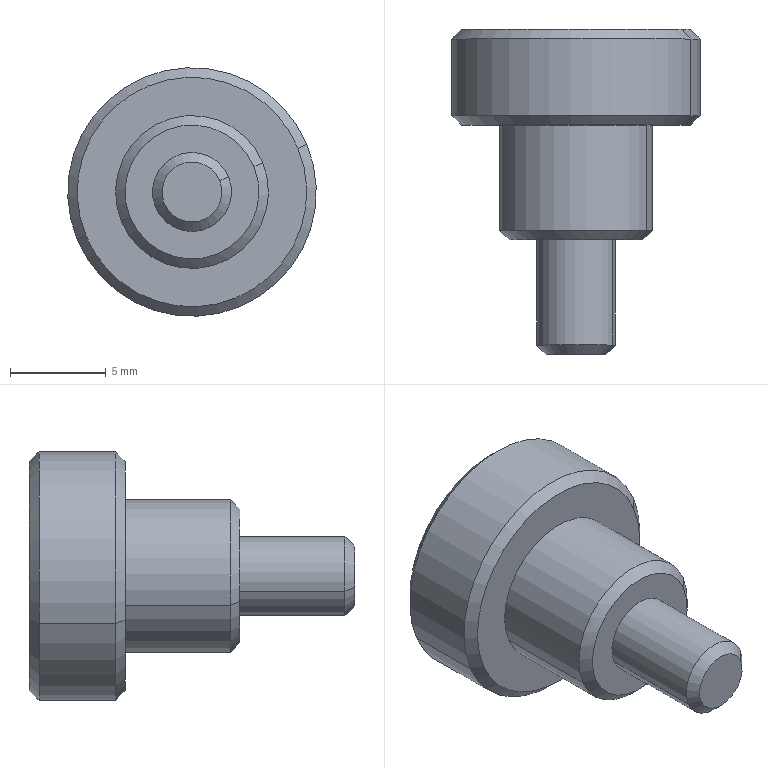Component | SolidWorks | BearingLiftingModule-1_CylinderLiftingModule-1_CHEN123-AA-26-1 | 1 solid | 18 faces | box 13 x 17 x 13 mm | volume 1031 mm3 | cone 8 | cylinder 6 | plane 4 | commonest cylinder face diameters 4.134 x2 8 x2 13 x2
build123d program:
from build123d import *

# Parameters (mm, degrees)
SKETCH1_R           = 6.5
BOSS_EXTRUDE1_DEPTH = 5
SKETCH2_R           = 4
BOSS_EXTRUDE2_DEPTH = 6
SKETCH3_R           = 2.067
BOSS_EXTRUDE3_DEPTH = 6
CHAMFER1_SIZE       = 0.5


with BuildPart() as part:
    # Sketch1 → Boss-Extrude1 (new body)
    with BuildSketch(Plane.XY):
        Circle(SKETCH1_R)
    extrude(amount=BOSS_EXTRUDE1_DEPTH)

    # Sketch2 → Boss-Extrude2 (add)
    with BuildSketch(Plane.XY.offset(5)):
        Circle(SKETCH2_R)
    extrude(amount=BOSS_EXTRUDE2_DEPTH)

    # Sketch3 → Boss-Extrude3 (add)
    with BuildSketch(Plane.XY.offset(11)):
        Circle(SKETCH3_R)
    extrude(amount=BOSS_EXTRUDE3_DEPTH)

    # Chamfer1
    chamfer1_edges = [part.edges().sort_by_distance(p)[0] for p in [
        (-2.067, 0, 17),
        (-6.5, 0, 0),
        (-6.5, 0, 5),
        (-4, 0, 11),
    ]]
    chamfer(chamfer1_edges, length=CHAMFER1_SIZE)


solid = part.part

# Placed as in the assembly
solid = solid.moved(Location((69.999, -35.699, 30), (90, 0, 0)))
STEP:
#1=COLOUR_RGB('',0.7922,0.8196,0.9333);
#2=FILL_AREA_STYLE_COLOUR('',#1);
#3=FILL_AREA_STYLE('',(#2));
#4=SURFACE_STYLE_FILL_AREA(#3);
#5=SURFACE_SIDE_STYLE('',(#4));
#6=SURFACE_STYLE_USAGE(.BOTH.,#5);
#7=PRESENTATION_STYLE_ASSIGNMENT((#6));
#8=CARTESIAN_POINT('',(2.538,-1.405,1.091));
#9=VERTEX_POINT('',#8);
#10=CARTESIAN_POINT('',(2.974,-1.405,1.271));
#11=VERTEX_POINT('',#10);
#12=CARTESIAN_POINT('',(2.756,-1.405,1.181));
#13=DIRECTION('',(-0.,1.,-0.));
#14=DIRECTION('',(0.9242,0.,0.3818));
#15=AXIS2_PLACEMENT_3D('',#12,#13,#14);
#16=CIRCLE('',#15,0.2362);
#17=EDGE_CURVE('',#9,#11,#16,.T.);
#18=ORIENTED_EDGE('',*,*,#17,.F.);
#19=CARTESIAN_POINT('',(2.519,-1.425,1.083));
#20=VERTEX_POINT('',#19);
#21=CARTESIAN_POINT('',(2.519,-1.425,1.083));
#22=DIRECTION('',(-0.6535,-0.7071,-0.27));
#23=VECTOR('',#22,39.37);
#24=LINE('',#21,#23);
#25=EDGE_CURVE('',#9,#20,#24,.T.);
#26=ORIENTED_EDGE('',*,*,#25,.T.);
#27=CARTESIAN_POINT('',(2.992,-1.425,1.279));
#28=VERTEX_POINT('',#27);
#29=CARTESIAN_POINT('',(2.756,-1.425,1.181));
#30=DIRECTION('',(0.,-1.,0.));
#31=DIRECTION('',(0.9242,0.,0.3818));
#32=AXIS2_PLACEMENT_3D('',#29,#30,#31);
#33=CIRCLE('',#32,0.2559);
#34=EDGE_CURVE('',#28,#20,#33,.T.);
#35=ORIENTED_EDGE('',*,*,#34,.F.);
#36=CARTESIAN_POINT('',(2.992,-1.425,1.279));
#37=DIRECTION('',(0.6535,-0.7071,0.27));
#38=VECTOR('',#37,39.37);
#39=LINE('',#36,#38);
#40=EDGE_CURVE('',#11,#28,#39,.T.);
#41=ORIENTED_EDGE('',*,*,#40,.F.);
#42=EDGE_LOOP('',(#18,#26,#35,#41));
#43=FACE_OUTER_BOUND('',#42,.T.);
#44=CARTESIAN_POINT('',(2.756,-1.425,1.181));
#45=DIRECTION('',(0.,-1.,0.));
#46=DIRECTION('',(0.9242,0.,0.3818));
#47=AXIS2_PLACEMENT_3D('',#44,#45,#46);
#48=CONICAL_SURFACE('',#47,0.2559,0.7854);
#49=ADVANCED_FACE('',(#43),#48,.T.);
#50=CARTESIAN_POINT('',(2.813,-2.075,1.205));
#51=VERTEX_POINT('',#50);
#52=CARTESIAN_POINT('',(2.699,-2.075,1.158));
#53=VERTEX_POINT('',#52);
#54=CARTESIAN_POINT('',(2.756,-2.075,1.181));
#55=DIRECTION('',(0.,-1.,0.));
#56=DIRECTION('',(0.9242,0.,0.3818));
#57=AXIS2_PLACEMENT_3D('',#54,#55,#56);
#58=CIRCLE('',#57,0.06169);
#59=EDGE_CURVE('',#51,#53,#58,.T.);
#60=ORIENTED_EDGE('',*,*,#59,.F.);
#61=CARTESIAN_POINT('',(2.831,-2.055,1.212));
#62=VERTEX_POINT('',#61);
#63=CARTESIAN_POINT('',(2.813,-2.075,1.205));
#64=DIRECTION('',(0.6535,0.7071,0.27));
#65=VECTOR('',#64,39.37);
#66=LINE('',#63,#65);
#67=EDGE_CURVE('',#51,#62,#66,.T.);
#68=ORIENTED_EDGE('',*,*,#67,.T.);
#69=CARTESIAN_POINT('',(2.681,-2.055,1.15));
#70=VERTEX_POINT('',#69);
#71=CARTESIAN_POINT('',(2.756,-2.055,1.181));
#72=DIRECTION('',(-0.,1.,-0.));
#73=DIRECTION('',(0.9242,0.,0.3818));
#74=AXIS2_PLACEMENT_3D('',#71,#72,#73);
#75=CIRCLE('',#74,0.08138);
#76=EDGE_CURVE('',#70,#62,#75,.T.);
#77=ORIENTED_EDGE('',*,*,#76,.F.);
#78=CARTESIAN_POINT('',(2.699,-2.075,1.158));
#79=DIRECTION('',(-0.6535,0.7071,-0.27));
#80=VECTOR('',#79,39.37);
#81=LINE('',#78,#80);
#82=EDGE_CURVE('',#53,#70,#81,.T.);
#83=ORIENTED_EDGE('',*,*,#82,.F.);
#84=EDGE_LOOP('',(#60,#68,#77,#83));
#85=FACE_OUTER_BOUND('',#84,.T.);
#86=CARTESIAN_POINT('',(2.756,-2.075,1.181));
#87=DIRECTION('',(-0.,1.,-0.));
#88=DIRECTION('',(-0.9242,0.,-0.3818));
#89=AXIS2_PLACEMENT_3D('',#86,#87,#88);
#90=CONICAL_SURFACE('',#89,0.06169,0.7854);
#91=ADVANCED_FACE('',(#85),#90,.T.);
#92=CARTESIAN_POINT('',(2.883,-1.839,1.234));
#93=VERTEX_POINT('',#92);
#94=CARTESIAN_POINT('',(2.629,-1.839,1.128));
#95=VERTEX_POINT('',#94);
#96=CARTESIAN_POINT('',(2.756,-1.839,1.181));
#97=DIRECTION('',(0.,-1.,0.));
#98=DIRECTION('',(0.9242,0.,0.3818));
#99=AXIS2_PLACEMENT_3D('',#96,#97,#98);
#100=CIRCLE('',#99,0.1378);
#101=EDGE_CURVE('',#93,#95,#100,.T.);
#102=ORIENTED_EDGE('',*,*,#101,.F.);
#103=CARTESIAN_POINT('',(2.901,-1.819,1.241));
#104=VERTEX_POINT('',#103);
#105=CARTESIAN_POINT('',(2.883,-1.839,1.234));
#106=DIRECTION('',(0.6535,0.7071,0.27));
#107=VECTOR('',#106,39.37);
#108=LINE('',#105,#107);
#109=EDGE_CURVE('',#93,#104,#108,.T.);
#110=ORIENTED_EDGE('',*,*,#109,.T.);
#111=CARTESIAN_POINT('',(2.61,-1.819,1.121));
#112=VERTEX_POINT('',#111);
#113=CARTESIAN_POINT('',(2.756,-1.819,1.181));
#114=DIRECTION('',(-0.,1.,-0.));
#115=DIRECTION('',(0.9242,0.,0.3818));
#116=AXIS2_PLACEMENT_3D('',#113,#114,#115);
#117=CIRCLE('',#116,0.1575);
#118=EDGE_CURVE('',#112,#104,#117,.T.);
#119=ORIENTED_EDGE('',*,*,#118,.F.);
#120=CARTESIAN_POINT('',(2.629,-1.839,1.128));
#121=DIRECTION('',(-0.6535,0.7071,-0.27));
#122=VECTOR('',#121,39.37);
#123=LINE('',#120,#122);
#124=EDGE_CURVE('',#95,#112,#123,.T.);
#125=ORIENTED_EDGE('',*,*,#124,.F.);
#126=EDGE_LOOP('',(#102,#110,#119,#125));
#127=FACE_OUTER_BOUND('',#126,.T.);
#128=CARTESIAN_POINT('',(2.756,-1.839,1.181));
#129=DIRECTION('',(-0.,1.,-0.));
#130=DIRECTION('',(-0.9242,0.,-0.3818));
#131=AXIS2_PLACEMENT_3D('',#128,#129,#130);
#132=CONICAL_SURFACE('',#131,0.1378,0.7854);
#133=ADVANCED_FACE('',(#127),#132,.T.);
#134=CARTESIAN_POINT('',(2.974,-1.602,1.271));
#135=VERTEX_POINT('',#134);
#136=CARTESIAN_POINT('',(2.538,-1.602,1.091));
#137=VERTEX_POINT('',#136);
#138=CARTESIAN_POINT('',(2.756,-1.602,1.181));
#139=DIRECTION('',(0.,-1.,0.));
#140=DIRECTION('',(0.9242,0.,0.3818));
#141=AXIS2_PLACEMENT_3D('',#138,#139,#140);
#142=CIRCLE('',#141,0.2362);
#143=EDGE_CURVE('',#135,#137,#142,.T.);
#144=ORIENTED_EDGE('',*,*,#143,.F.);
#145=CARTESIAN_POINT('',(2.992,-1.583,1.279));
#146=VERTEX_POINT('',#145);
#147=CARTESIAN_POINT('',(2.974,-1.602,1.271));
#148=DIRECTION('',(0.6535,0.7071,0.27));
#149=VECTOR('',#148,39.37);
#150=LINE('',#147,#149);
#151=EDGE_CURVE('',#135,#146,#150,.T.);
#152=ORIENTED_EDGE('',*,*,#151,.T.);
#153=CARTESIAN_POINT('',(2.519,-1.583,1.083));
#154=VERTEX_POINT('',#153);
#155=CARTESIAN_POINT('',(2.756,-1.583,1.181));
#156=DIRECTION('',(-0.,1.,-0.));
#157=DIRECTION('',(0.9242,0.,0.3818));
#158=AXIS2_PLACEMENT_3D('',#155,#156,#157);
#159=CIRCLE('',#158,0.2559);
#160=EDGE_CURVE('',#154,#146,#159,.T.);
#161=ORIENTED_EDGE('',*,*,#160,.F.);
#162=CARTESIAN_POINT('',(2.538,-1.602,1.091));
#163=DIRECTION('',(-0.6535,0.7071,-0.27));
#164=VECTOR('',#163,39.37);
#165=LINE('',#162,#164);
#166=EDGE_CURVE('',#137,#154,#165,.T.);
#167=ORIENTED_EDGE('',*,*,#166,.F.);
#168=EDGE_LOOP('',(#144,#152,#161,#167));
#169=FACE_OUTER_BOUND('',#168,.T.);
#170=CARTESIAN_POINT('',(2.756,-1.602,1.181));
#171=DIRECTION('',(-0.,1.,-0.));
#172=DIRECTION('',(-0.9242,0.,-0.3818));
#173=AXIS2_PLACEMENT_3D('',#170,#171,#172);
#174=CONICAL_SURFACE('',#173,0.2362,0.7854);
#175=ADVANCED_FACE('',(#169),#174,.T.);
#176=ORIENTED_EDGE('',*,*,#76,.T.);
#177=CARTESIAN_POINT('',(2.831,-1.839,1.212));
#178=VERTEX_POINT('',#177);
#179=CARTESIAN_POINT('',(2.831,-2.075,1.212));
#180=DIRECTION('',(-0.,1.,-0.));
#181=VECTOR('',#180,39.37);
#182=LINE('',#179,#181);
#183=EDGE_CURVE('',#62,#178,#182,.T.);
#184=ORIENTED_EDGE('',*,*,#183,.T.);
#185=CARTESIAN_POINT('',(2.681,-1.839,1.15));
#186=VERTEX_POINT('',#185);
#187=CARTESIAN_POINT('',(2.756,-1.839,1.181));
#188=DIRECTION('',(0.,-1.,0.));
#189=DIRECTION('',(0.9242,0.,0.3818));
#190=AXIS2_PLACEMENT_3D('',#187,#188,#189);
#191=CIRCLE('',#190,0.08138);
#192=EDGE_CURVE('',#178,#186,#191,.T.);
#193=ORIENTED_EDGE('',*,*,#192,.T.);
#194=CARTESIAN_POINT('',(2.681,-2.075,1.15));
#195=DIRECTION('',(-0.,1.,-0.));
#196=VECTOR('',#195,39.37);
#197=LINE('',#194,#196);
#198=EDGE_CURVE('',#70,#186,#197,.T.);
#199=ORIENTED_EDGE('',*,*,#198,.F.);
#200=EDGE_LOOP('',(#176,#184,#193,#199));
#201=FACE_OUTER_BOUND('',#200,.T.);
#202=CARTESIAN_POINT('',(2.756,-2.075,1.181));
#203=DIRECTION('',(-0.,1.,-0.));
#204=DIRECTION('',(-0.9242,0.,-0.3818));
#205=AXIS2_PLACEMENT_3D('',#202,#203,#204);
#206=CYLINDRICAL_SURFACE('',#205,0.08138);
#207=ADVANCED_FACE('',(#201),#206,.T.);
#208=ORIENTED_EDGE('',*,*,#118,.T.);
#209=CARTESIAN_POINT('',(2.901,-1.602,1.241));
#210=VERTEX_POINT('',#209);
#211=CARTESIAN_POINT('',(2.901,-1.839,1.241));
#212=DIRECTION('',(-0.,1.,-0.));
#213=VECTOR('',#212,39.37);
#214=LINE('',#211,#213);
#215=EDGE_CURVE('',#104,#210,#214,.T.);
#216=ORIENTED_EDGE('',*,*,#215,.T.);
#217=CARTESIAN_POINT('',(2.61,-1.602,1.121));
#218=VERTEX_POINT('',#217);
#219=CARTESIAN_POINT('',(2.756,-1.602,1.181));
#220=DIRECTION('',(0.,-1.,0.));
#221=DIRECTION('',(0.9242,0.,0.3818));
#222=AXIS2_PLACEMENT_3D('',#219,#220,#221);
#223=CIRCLE('',#222,0.1575);
#224=EDGE_CURVE('',#210,#218,#223,.T.);
#225=ORIENTED_EDGE('',*,*,#224,.T.);
#226=CARTESIAN_POINT('',(2.61,-1.839,1.121));
#227=DIRECTION('',(-0.,1.,-0.));
#228=VECTOR('',#227,39.37);
#229=LINE('',#226,#228);
#230=EDGE_CURVE('',#112,#218,#229,.T.);
#231=ORIENTED_EDGE('',*,*,#230,.F.);
#232=EDGE_LOOP('',(#208,#216,#225,#231));
#233=FACE_OUTER_BOUND('',#232,.T.);
#234=CARTESIAN_POINT('',(2.756,-1.839,1.181));
#235=DIRECTION('',(-0.,1.,-0.));
#236=DIRECTION('',(-0.9242,0.,-0.3818));
#237=AXIS2_PLACEMENT_3D('',#234,#235,#236);
#238=CYLINDRICAL_SURFACE('',#237,0.1575);
#239=ADVANCED_FACE('',(#233),#238,.T.);
#240=ORIENTED_EDGE('',*,*,#160,.T.);
#241=CARTESIAN_POINT('',(2.992,-1.602,1.279));
#242=DIRECTION('',(-0.,1.,-0.));
#243=VECTOR('',#242,39.37);
#244=LINE('',#241,#243);
#245=EDGE_CURVE('',#146,#28,#244,.T.);
#246=ORIENTED_EDGE('',*,*,#245,.T.);
#247=ORIENTED_EDGE('',*,*,#34,.T.);
#248=CARTESIAN_POINT('',(2.519,-1.602,1.083));
#249=DIRECTION('',(-0.,1.,-0.));
#250=VECTOR('',#249,39.37);
#251=LINE('',#248,#250);
#252=EDGE_CURVE('',#154,#20,#251,.T.);
#253=ORIENTED_EDGE('',*,*,#252,.F.);
#254=EDGE_LOOP('',(#240,#246,#247,#253));
#255=FACE_OUTER_BOUND('',#254,.T.);
#256=CARTESIAN_POINT('',(2.756,-1.602,1.181));
#257=DIRECTION('',(-0.,1.,-0.));
#258=DIRECTION('',(-0.9242,0.,-0.3818));
#259=AXIS2_PLACEMENT_3D('',#256,#257,#258);
#260=CYLINDRICAL_SURFACE('',#259,0.2559);
#261=ADVANCED_FACE('',(#255),#260,.T.);
#262=ORIENTED_EDGE('',*,*,#245,.F.);
#263=CARTESIAN_POINT('',(2.756,-1.583,1.181));
#264=DIRECTION('',(-0.,1.,-0.));
#265=DIRECTION('',(0.9242,0.,0.3818));
#266=AXIS2_PLACEMENT_3D('',#263,#264,#265);
#267=CIRCLE('',#266,0.2559);
#268=EDGE_CURVE('',#146,#154,#267,.T.);
#269=ORIENTED_EDGE('',*,*,#268,.T.);
#270=ORIENTED_EDGE('',*,*,#252,.T.);
#271=CARTESIAN_POINT('',(2.756,-1.425,1.181));
#272=DIRECTION('',(0.,-1.,0.));
#273=DIRECTION('',(0.9242,0.,0.3818));
#274=AXIS2_PLACEMENT_3D('',#271,#272,#273);
#275=CIRCLE('',#274,0.2559);
#276=EDGE_CURVE('',#20,#28,#275,.T.);
#277=ORIENTED_EDGE('',*,*,#276,.T.);
#278=EDGE_LOOP('',(#262,#269,#270,#277));
#279=FACE_OUTER_BOUND('',#278,.T.);
#280=CARTESIAN_POINT('',(2.756,-1.602,1.181));
#281=DIRECTION('',(-0.,1.,-0.));
#282=DIRECTION('',(-0.9242,0.,-0.3818));
#283=AXIS2_PLACEMENT_3D('',#280,#281,#282);
#284=CYLINDRICAL_SURFACE('',#283,0.2559);
#285=ADVANCED_FACE('',(#279),#284,.T.);
#286=CARTESIAN_POINT('',(2.756,-1.602,1.181));
#287=DIRECTION('',(0.,-1.,0.));
#288=DIRECTION('',(0.9242,0.,0.3818));
#289=AXIS2_PLACEMENT_3D('',#286,#287,#288);
#290=CIRCLE('',#289,0.2362);
#291=EDGE_CURVE('',#137,#135,#290,.T.);
#292=ORIENTED_EDGE('',*,*,#291,.T.);
#293=ORIENTED_EDGE('',*,*,#143,.T.);
#294=EDGE_LOOP('',(#292,#293));
#295=FACE_OUTER_BOUND('',#294,.T.);
#296=CARTESIAN_POINT('',(2.756,-1.602,1.181));
#297=DIRECTION('',(0.,-1.,0.));
#298=DIRECTION('',(0.9242,0.,0.3818));
#299=AXIS2_PLACEMENT_3D('',#296,#297,#298);
#300=CIRCLE('',#299,0.1575);
#301=EDGE_CURVE('',#218,#210,#300,.T.);
#302=ORIENTED_EDGE('',*,*,#301,.F.);
#303=ORIENTED_EDGE('',*,*,#224,.F.);
#304=EDGE_LOOP('',(#302,#303));
#305=FACE_BOUND('',#304,.T.);
#306=CARTESIAN_POINT('',(2.756,-1.602,1.181));
#307=DIRECTION('',(-0.,-1.,0.));
#308=DIRECTION('',(0.9242,0.,0.3818));
#309=AXIS2_PLACEMENT_3D('',#306,#307,#308);
#310=PLANE('',#309);
#311=ADVANCED_FACE('',(#295,#305),#310,.T.);
#312=CARTESIAN_POINT('',(2.756,-1.405,1.181));
#313=DIRECTION('',(-0.,1.,-0.));
#314=DIRECTION('',(0.9242,0.,0.3818));
#315=AXIS2_PLACEMENT_3D('',#312,#313,#314);
#316=CIRCLE('',#315,0.2362);
#317=EDGE_CURVE('',#11,#9,#316,.T.);
#318=ORIENTED_EDGE('',*,*,#317,.T.);
#319=ORIENTED_EDGE('',*,*,#17,.T.);
#320=EDGE_LOOP('',(#318,#319));
#321=FACE_OUTER_BOUND('',#320,.T.);
#322=CARTESIAN_POINT('',(2.756,-1.405,1.181));
#323=DIRECTION('',(-0.,-1.,0.));
#324=DIRECTION('',(0.9242,0.,0.3818));
#325=AXIS2_PLACEMENT_3D('',#322,#323,#324);
#326=PLANE('',#325);
#327=ADVANCED_FACE('',(#321),#326,.F.);
#328=ORIENTED_EDGE('',*,*,#215,.F.);
#329=CARTESIAN_POINT('',(2.756,-1.819,1.181));
#330=DIRECTION('',(-0.,1.,-0.));
#331=DIRECTION('',(0.9242,0.,0.3818));
#332=AXIS2_PLACEMENT_3D('',#329,#330,#331);
#333=CIRCLE('',#332,0.1575);
#334=EDGE_CURVE('',#104,#112,#333,.T.);
#335=ORIENTED_EDGE('',*,*,#334,.T.);
#336=ORIENTED_EDGE('',*,*,#230,.T.);
#337=ORIENTED_EDGE('',*,*,#301,.T.);
#338=EDGE_LOOP('',(#328,#335,#336,#337));
#339=FACE_OUTER_BOUND('',#338,.T.);
#340=CARTESIAN_POINT('',(2.756,-1.839,1.181));
#341=DIRECTION('',(-0.,1.,-0.));
#342=DIRECTION('',(-0.9242,0.,-0.3818));
#343=AXIS2_PLACEMENT_3D('',#340,#341,#342);
#344=CYLINDRICAL_SURFACE('',#343,0.1575);
#345=ADVANCED_FACE('',(#339),#344,.T.);
#346=CARTESIAN_POINT('',(2.756,-1.839,1.181));
#347=DIRECTION('',(0.,-1.,0.));
#348=DIRECTION('',(0.9242,0.,0.3818));
#349=AXIS2_PLACEMENT_3D('',#346,#347,#348);
#350=CIRCLE('',#349,0.1378);
#351=EDGE_CURVE('',#95,#93,#350,.T.);
#352=ORIENTED_EDGE('',*,*,#351,.T.);
#353=ORIENTED_EDGE('',*,*,#101,.T.);
#354=EDGE_LOOP('',(#352,#353));
#355=FACE_OUTER_BOUND('',#354,.T.);
#356=CARTESIAN_POINT('',(2.756,-1.839,1.181));
#357=DIRECTION('',(0.,-1.,0.));
#358=DIRECTION('',(0.9242,0.,0.3818));
#359=AXIS2_PLACEMENT_3D('',#356,#357,#358);
#360=CIRCLE('',#359,0.08138);
#361=EDGE_CURVE('',#186,#178,#360,.T.);
#362=ORIENTED_EDGE('',*,*,#361,.F.);
#363=ORIENTED_EDGE('',*,*,#192,.F.);
#364=EDGE_LOOP('',(#362,#363));
#365=FACE_BOUND('',#364,.T.);
#366=CARTESIAN_POINT('',(2.756,-1.839,1.181));
#367=DIRECTION('',(-0.,-1.,0.));
#368=DIRECTION('',(0.9242,0.,0.3818));
#369=AXIS2_PLACEMENT_3D('',#366,#367,#368);
#370=PLANE('',#369);
#371=ADVANCED_FACE('',(#355,#365),#370,.T.);
#372=ORIENTED_EDGE('',*,*,#183,.F.);
#373=CARTESIAN_POINT('',(2.756,-2.055,1.181));
#374=DIRECTION('',(-0.,1.,-0.));
#375=DIRECTION('',(0.9242,0.,0.3818));
#376=AXIS2_PLACEMENT_3D('',#373,#374,#375);
#377=CIRCLE('',#376,0.08138);
#378=EDGE_CURVE('',#62,#70,#377,.T.);
#379=ORIENTED_EDGE('',*,*,#378,.T.);
#380=ORIENTED_EDGE('',*,*,#198,.T.);
#381=ORIENTED_EDGE('',*,*,#361,.T.);
#382=EDGE_LOOP('',(#372,#379,#380,#381));
#383=FACE_OUTER_BOUND('',#382,.T.);
#384=CARTESIAN_POINT('',(2.756,-2.075,1.181));
#385=DIRECTION('',(-0.,1.,-0.));
#386=DIRECTION('',(-0.9242,0.,-0.3818));
#387=AXIS2_PLACEMENT_3D('',#384,#385,#386);
#388=CYLINDRICAL_SURFACE('',#387,0.08138);
#389=ADVANCED_FACE('',(#383),#388,.T.);
#390=CARTESIAN_POINT('',(2.756,-2.075,1.181));
#391=DIRECTION('',(0.,-1.,0.));
#392=DIRECTION('',(0.9242,0.,0.3818));
#393=AXIS2_PLACEMENT_3D('',#390,#391,#392);
#394=CIRCLE('',#393,0.06169);
#395=EDGE_CURVE('',#53,#51,#394,.T.);
#396=ORIENTED_EDGE('',*,*,#395,.T.);
#397=ORIENTED_EDGE('',*,*,#59,.T.);
#398=EDGE_LOOP('',(#396,#397));
#399=FACE_OUTER_BOUND('',#398,.T.);
#400=CARTESIAN_POINT('',(2.756,-2.075,1.181));
#401=DIRECTION('',(-0.,-1.,0.));
#402=DIRECTION('',(0.9242,0.,0.3818));
#403=AXIS2_PLACEMENT_3D('',#400,#401,#402);
#404=PLANE('',#403);
#405=ADVANCED_FACE('',(#399),#404,.T.);
#406=ORIENTED_EDGE('',*,*,#151,.F.);
#407=ORIENTED_EDGE('',*,*,#291,.F.);
#408=ORIENTED_EDGE('',*,*,#166,.T.);
#409=ORIENTED_EDGE('',*,*,#268,.F.);
#410=EDGE_LOOP('',(#406,#407,#408,#409));
#411=FACE_OUTER_BOUND('',#410,.T.);
#412=CARTESIAN_POINT('',(2.756,-1.602,1.181));
#413=DIRECTION('',(-0.,1.,-0.));
#414=DIRECTION('',(-0.9242,0.,-0.3818));
#415=AXIS2_PLACEMENT_3D('',#412,#413,#414);
#416=CONICAL_SURFACE('',#415,0.2362,0.7854);
#417=ADVANCED_FACE('',(#411),#416,.T.);
#418=ORIENTED_EDGE('',*,*,#109,.F.);
#419=ORIENTED_EDGE('',*,*,#351,.F.);
#420=ORIENTED_EDGE('',*,*,#124,.T.);
#421=ORIENTED_EDGE('',*,*,#334,.F.);
#422=EDGE_LOOP('',(#418,#419,#420,#421));
#423=FACE_OUTER_BOUND('',#422,.T.);
#424=CARTESIAN_POINT('',(2.756,-1.839,1.181));
#425=DIRECTION('',(-0.,1.,-0.));
#426=DIRECTION('',(-0.9242,0.,-0.3818));
#427=AXIS2_PLACEMENT_3D('',#424,#425,#426);
#428=CONICAL_SURFACE('',#427,0.1378,0.7854);
#429=ADVANCED_FACE('',(#423),#428,.T.);
#430=ORIENTED_EDGE('',*,*,#67,.F.);
#431=ORIENTED_EDGE('',*,*,#395,.F.);
#432=ORIENTED_EDGE('',*,*,#82,.T.);
#433=ORIENTED_EDGE('',*,*,#378,.F.);
#434=EDGE_LOOP('',(#430,#431,#432,#433));
#435=FACE_OUTER_BOUND('',#434,.T.);
#436=CARTESIAN_POINT('',(2.756,-2.075,1.181));
#437=DIRECTION('',(-0.,1.,-0.));
#438=DIRECTION('',(-0.9242,0.,-0.3818));
#439=AXIS2_PLACEMENT_3D('',#436,#437,#438);
#440=CONICAL_SURFACE('',#439,0.06169,0.7854);
#441=ADVANCED_FACE('',(#435),#440,.T.);
#442=ORIENTED_EDGE('',*,*,#25,.F.);
#443=ORIENTED_EDGE('',*,*,#317,.F.);
#444=ORIENTED_EDGE('',*,*,#40,.T.);
#445=ORIENTED_EDGE('',*,*,#276,.F.);
#446=EDGE_LOOP('',(#442,#443,#444,#445));
#447=FACE_OUTER_BOUND('',#446,.T.);
#448=CARTESIAN_POINT('',(2.756,-1.425,1.181));
#449=DIRECTION('',(0.,-1.,0.));
#450=DIRECTION('',(0.9242,0.,0.3818));
#451=AXIS2_PLACEMENT_3D('',#448,#449,#450);
#452=CONICAL_SURFACE('',#451,0.2559,0.7854);
#453=ADVANCED_FACE('',(#447),#452,.T.);
#454=CLOSED_SHELL('',(#49,#91,#133,#175,#207,#239,#261,#285,#311,#327,#345,#371,#389,#405,#417,#429,#441,#453));
#455=MANIFOLD_SOLID_BREP('',#454);
#456=STYLED_ITEM('',(#7),#455);
#457=PRESENTATION_LAYER_ASSIGNMENT('','',(#456));
#458=(LENGTH_UNIT()NAMED_UNIT(*)SI_UNIT($,.METRE.));
#459=LENGTH_MEASURE_WITH_UNIT(LENGTH_MEASURE(0.0254),#458);
#460=DIMENSIONAL_EXPONENTS(1.,0.,0.,0.,0.,0.,0.);
#461=(CONVERSION_BASED_UNIT('',#459)LENGTH_UNIT()NAMED_UNIT(#460));
#462=UNCERTAINTY_MEASURE_WITH_UNIT(LENGTH_MEASURE(0.00001),#461,'','');
#463=(NAMED_UNIT(*)PLANE_ANGLE_UNIT()SI_UNIT($,.RADIAN.));
#464=(NAMED_UNIT(*)SI_UNIT($,.STERADIAN.)SOLID_ANGLE_UNIT());
#465=(GEOMETRIC_REPRESENTATION_CONTEXT(3)GLOBAL_UNCERTAINTY_ASSIGNED_CONTEXT((#462))GLOBAL_UNIT_ASSIGNED_CONTEXT((#461,#463,#464))REPRESENTATION_CONTEXT('',''));
#466=MECHANICAL_DESIGN_GEOMETRIC_PRESENTATION_REPRESENTATION('',(#456),#465);
#467=CARTESIAN_POINT('',(0.,0.,0.));
#468=DIRECTION('',(0.,0.,1.));
#469=DIRECTION('',(1.,0.,0.));
#470=AXIS2_PLACEMENT_3D('',#467,#468,#469);
#471=(LENGTH_UNIT()NAMED_UNIT(*)SI_UNIT($,.METRE.));
#472=LENGTH_MEASURE_WITH_UNIT(LENGTH_MEASURE(0.0254),#471);
#473=DIMENSIONAL_EXPONENTS(1.,0.,0.,0.,0.,0.,0.);
#474=(CONVERSION_BASED_UNIT('',#472)LENGTH_UNIT()NAMED_UNIT(#473));
#475=UNCERTAINTY_MEASURE_WITH_UNIT(LENGTH_MEASURE(0.00001),#474,'','');
#476=(NAMED_UNIT(*)PLANE_ANGLE_UNIT()SI_UNIT($,.RADIAN.));
#477=(NAMED_UNIT(*)SI_UNIT($,.STERADIAN.)SOLID_ANGLE_UNIT());
#478=(GEOMETRIC_REPRESENTATION_CONTEXT(3)GLOBAL_UNCERTAINTY_ASSIGNED_CONTEXT((#475))GLOBAL_UNIT_ASSIGNED_CONTEXT((#474,#476,#477))REPRESENTATION_CONTEXT('',''));
#479=ADVANCED_BREP_SHAPE_REPRESENTATION('',(#455,#470),#478);